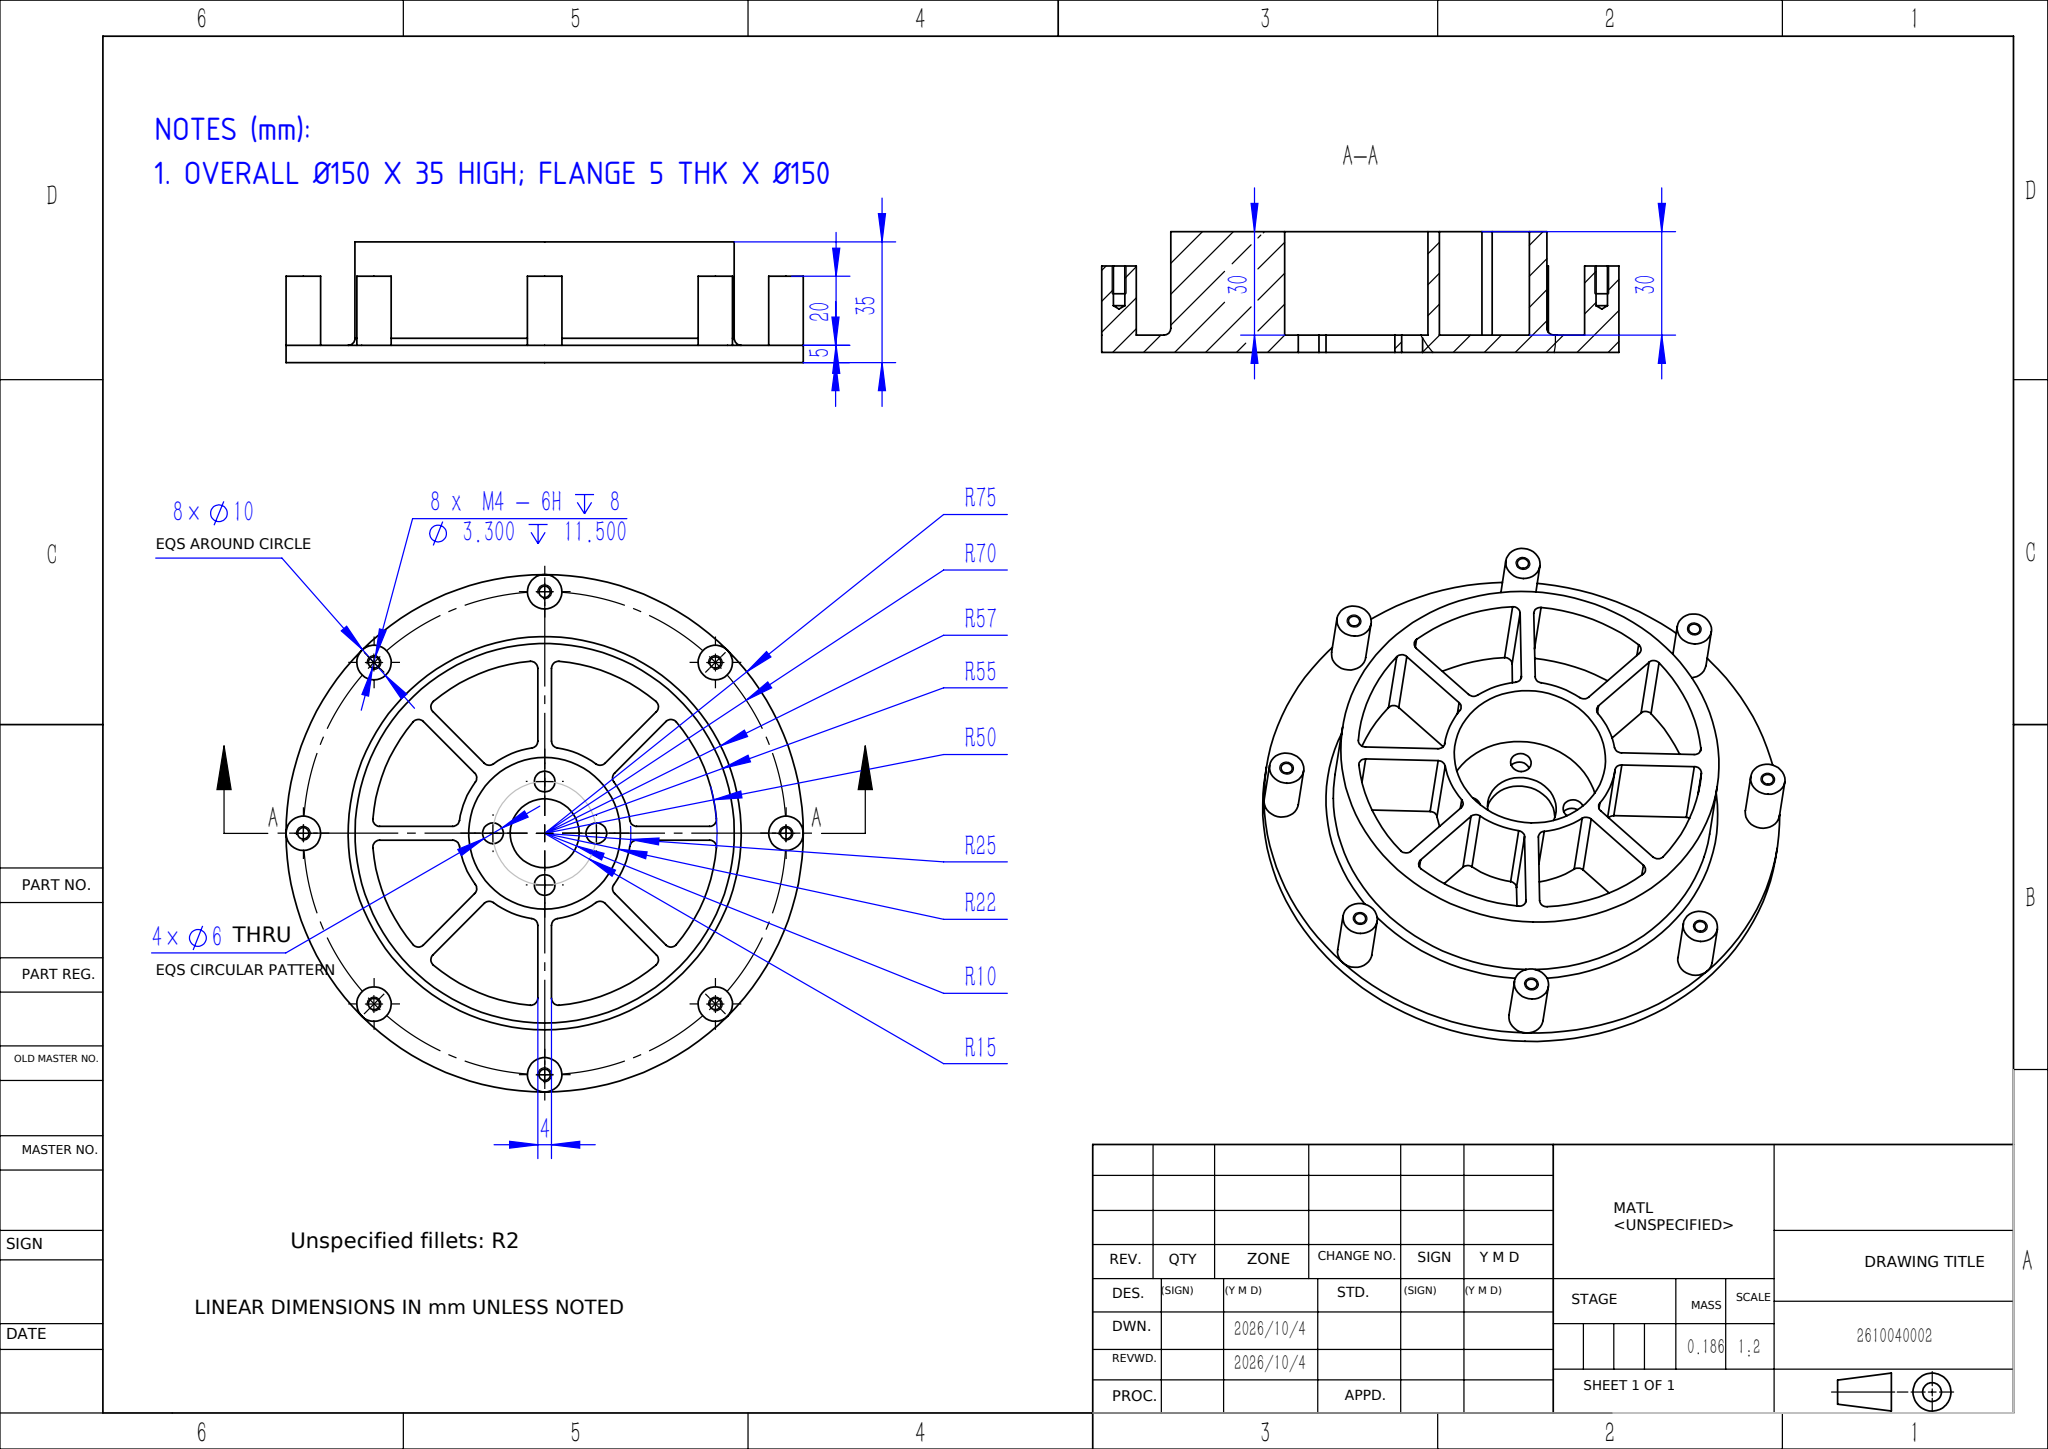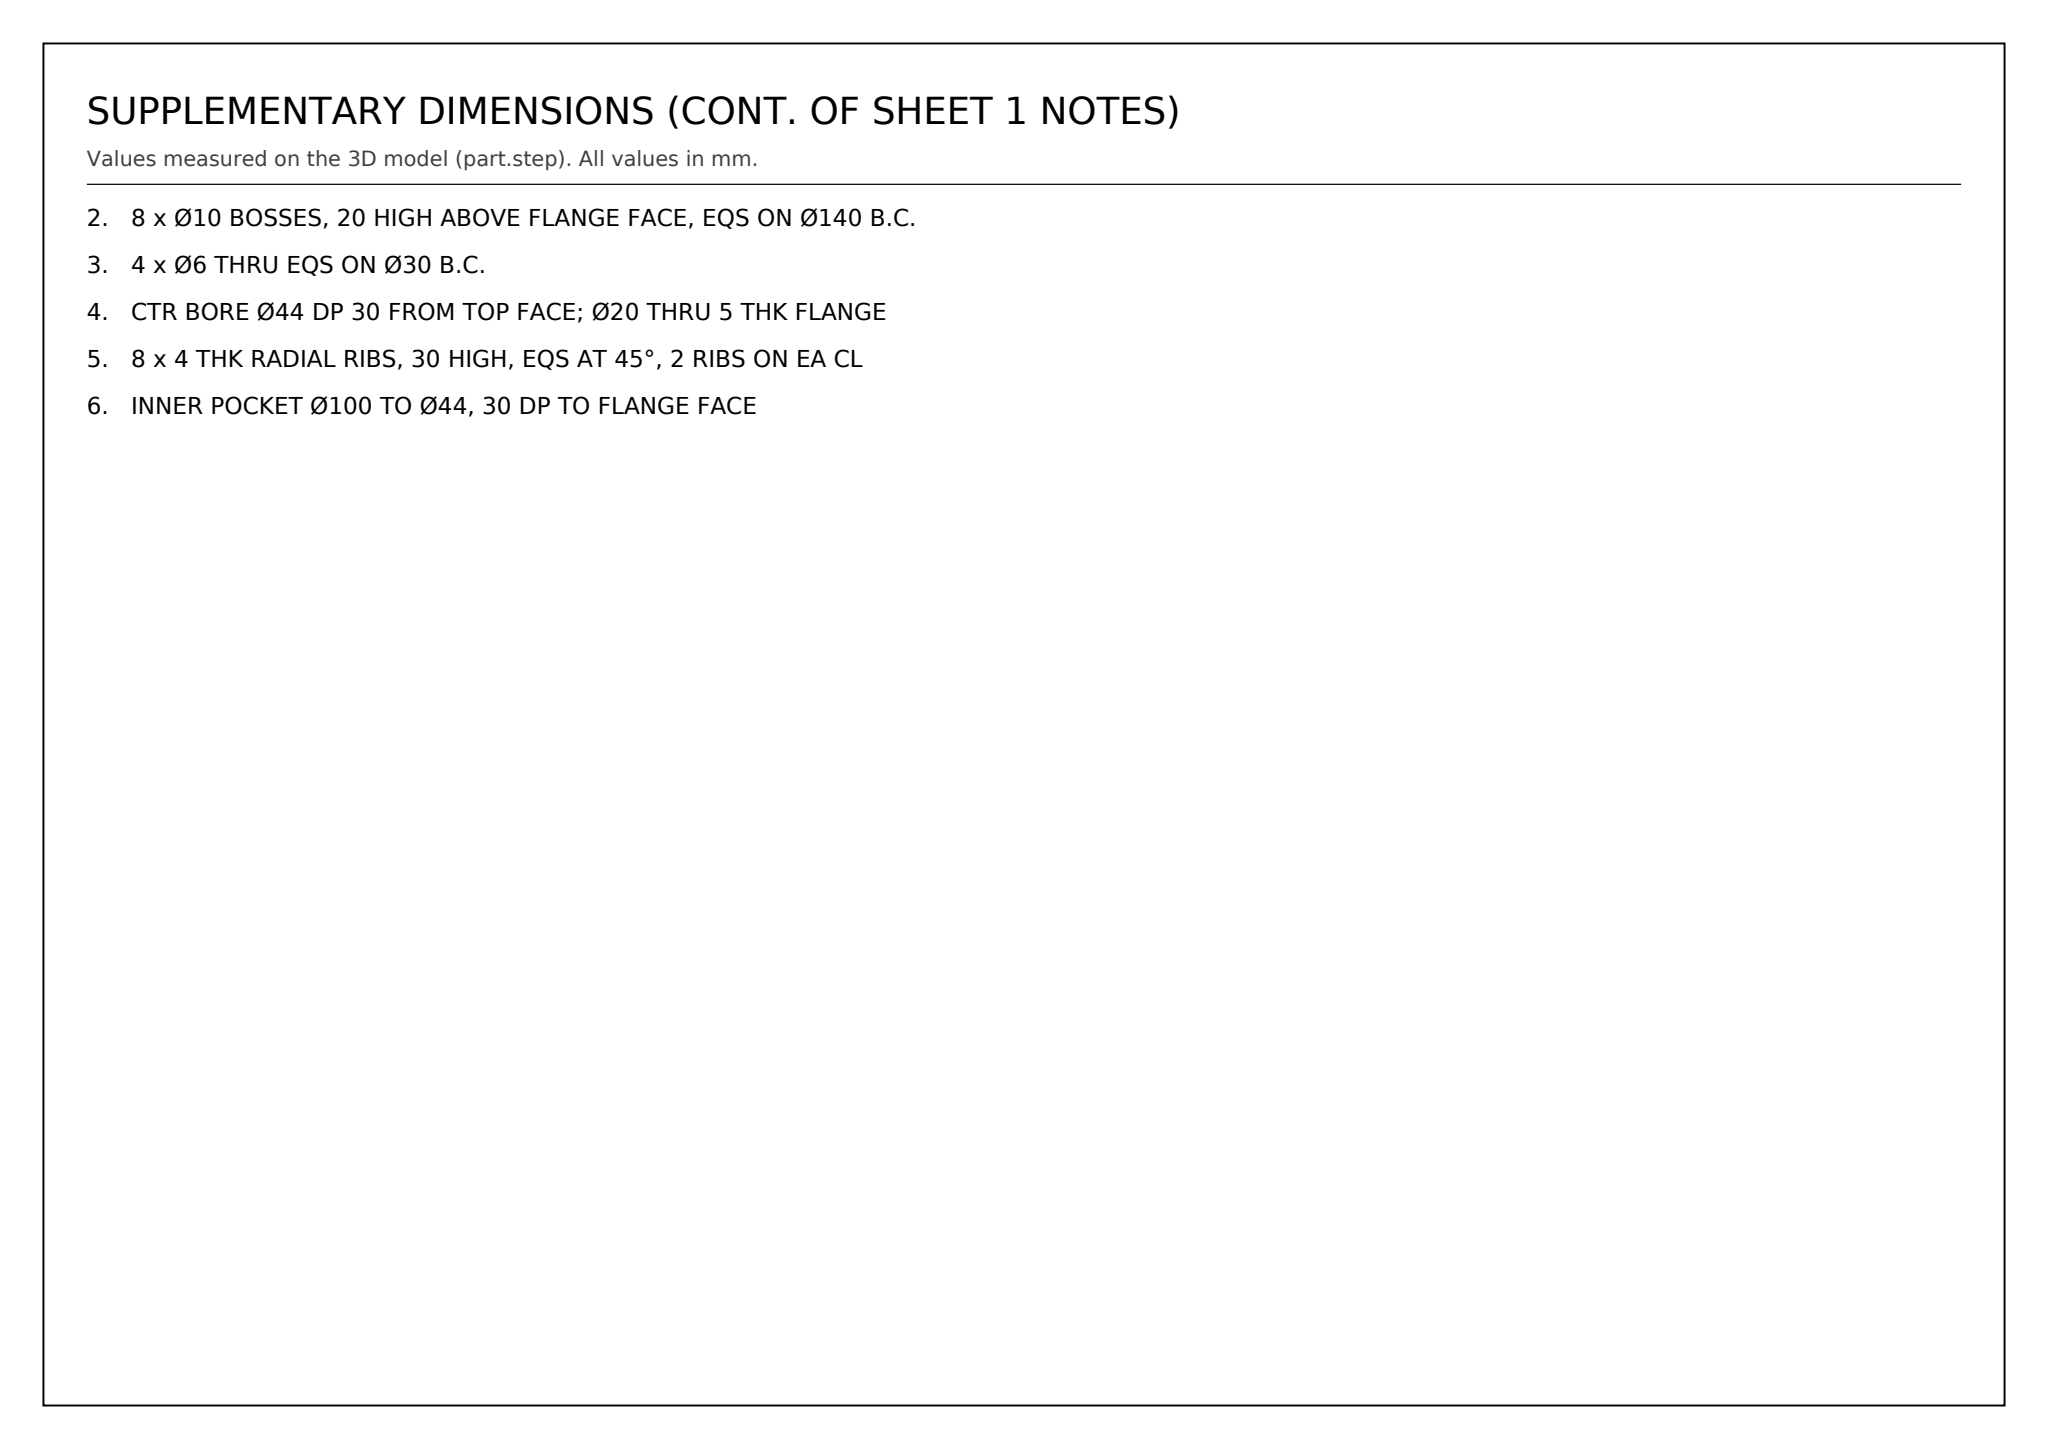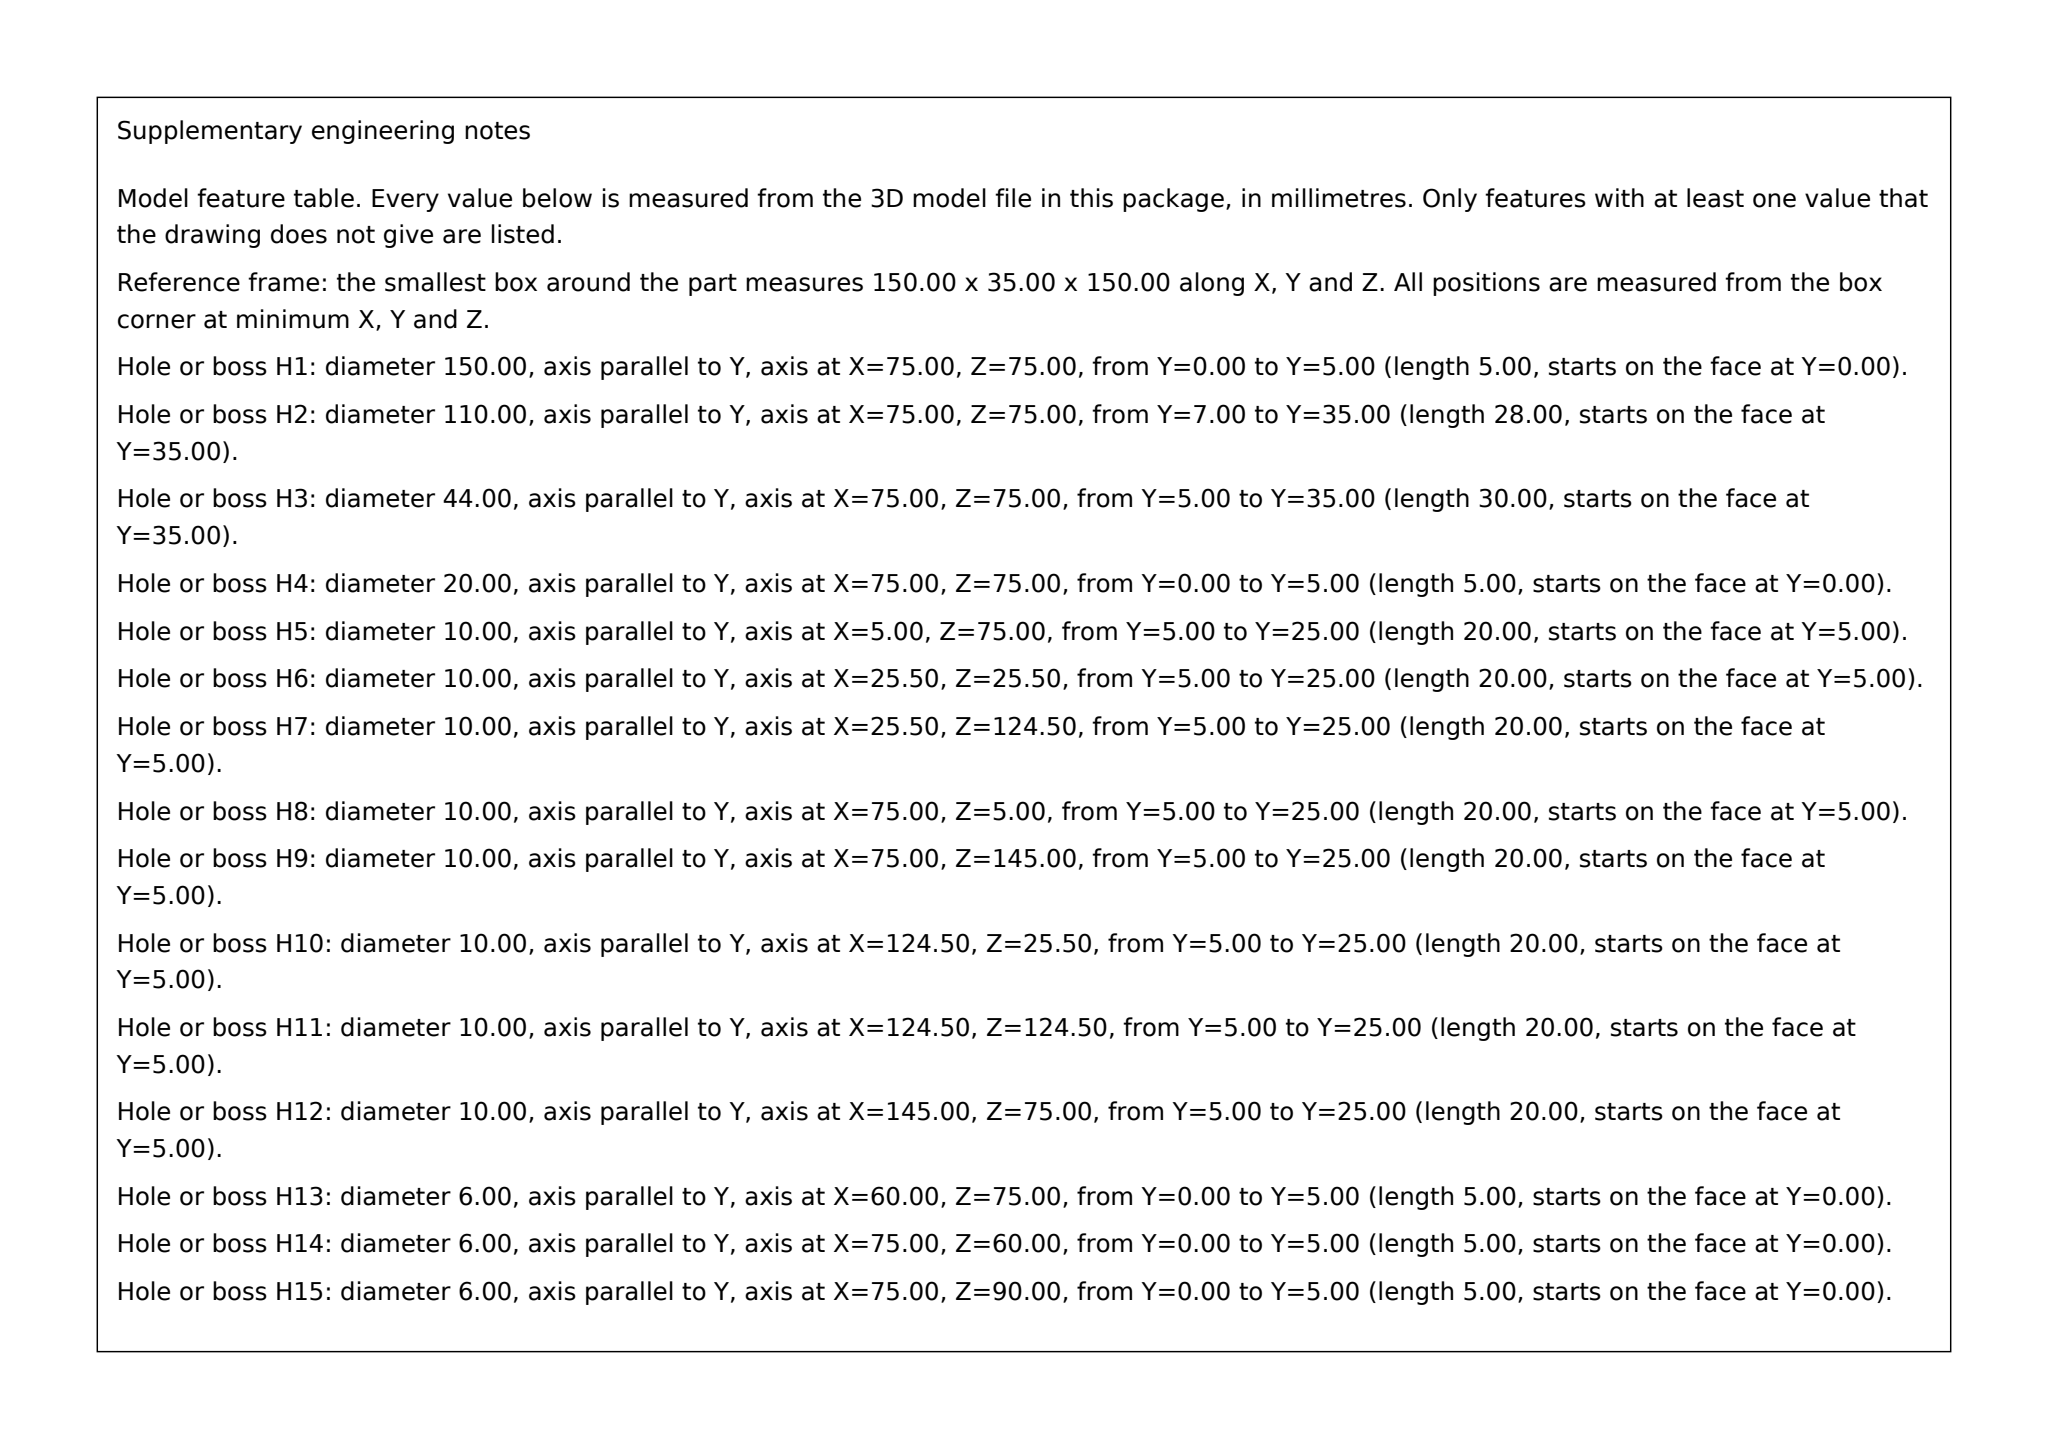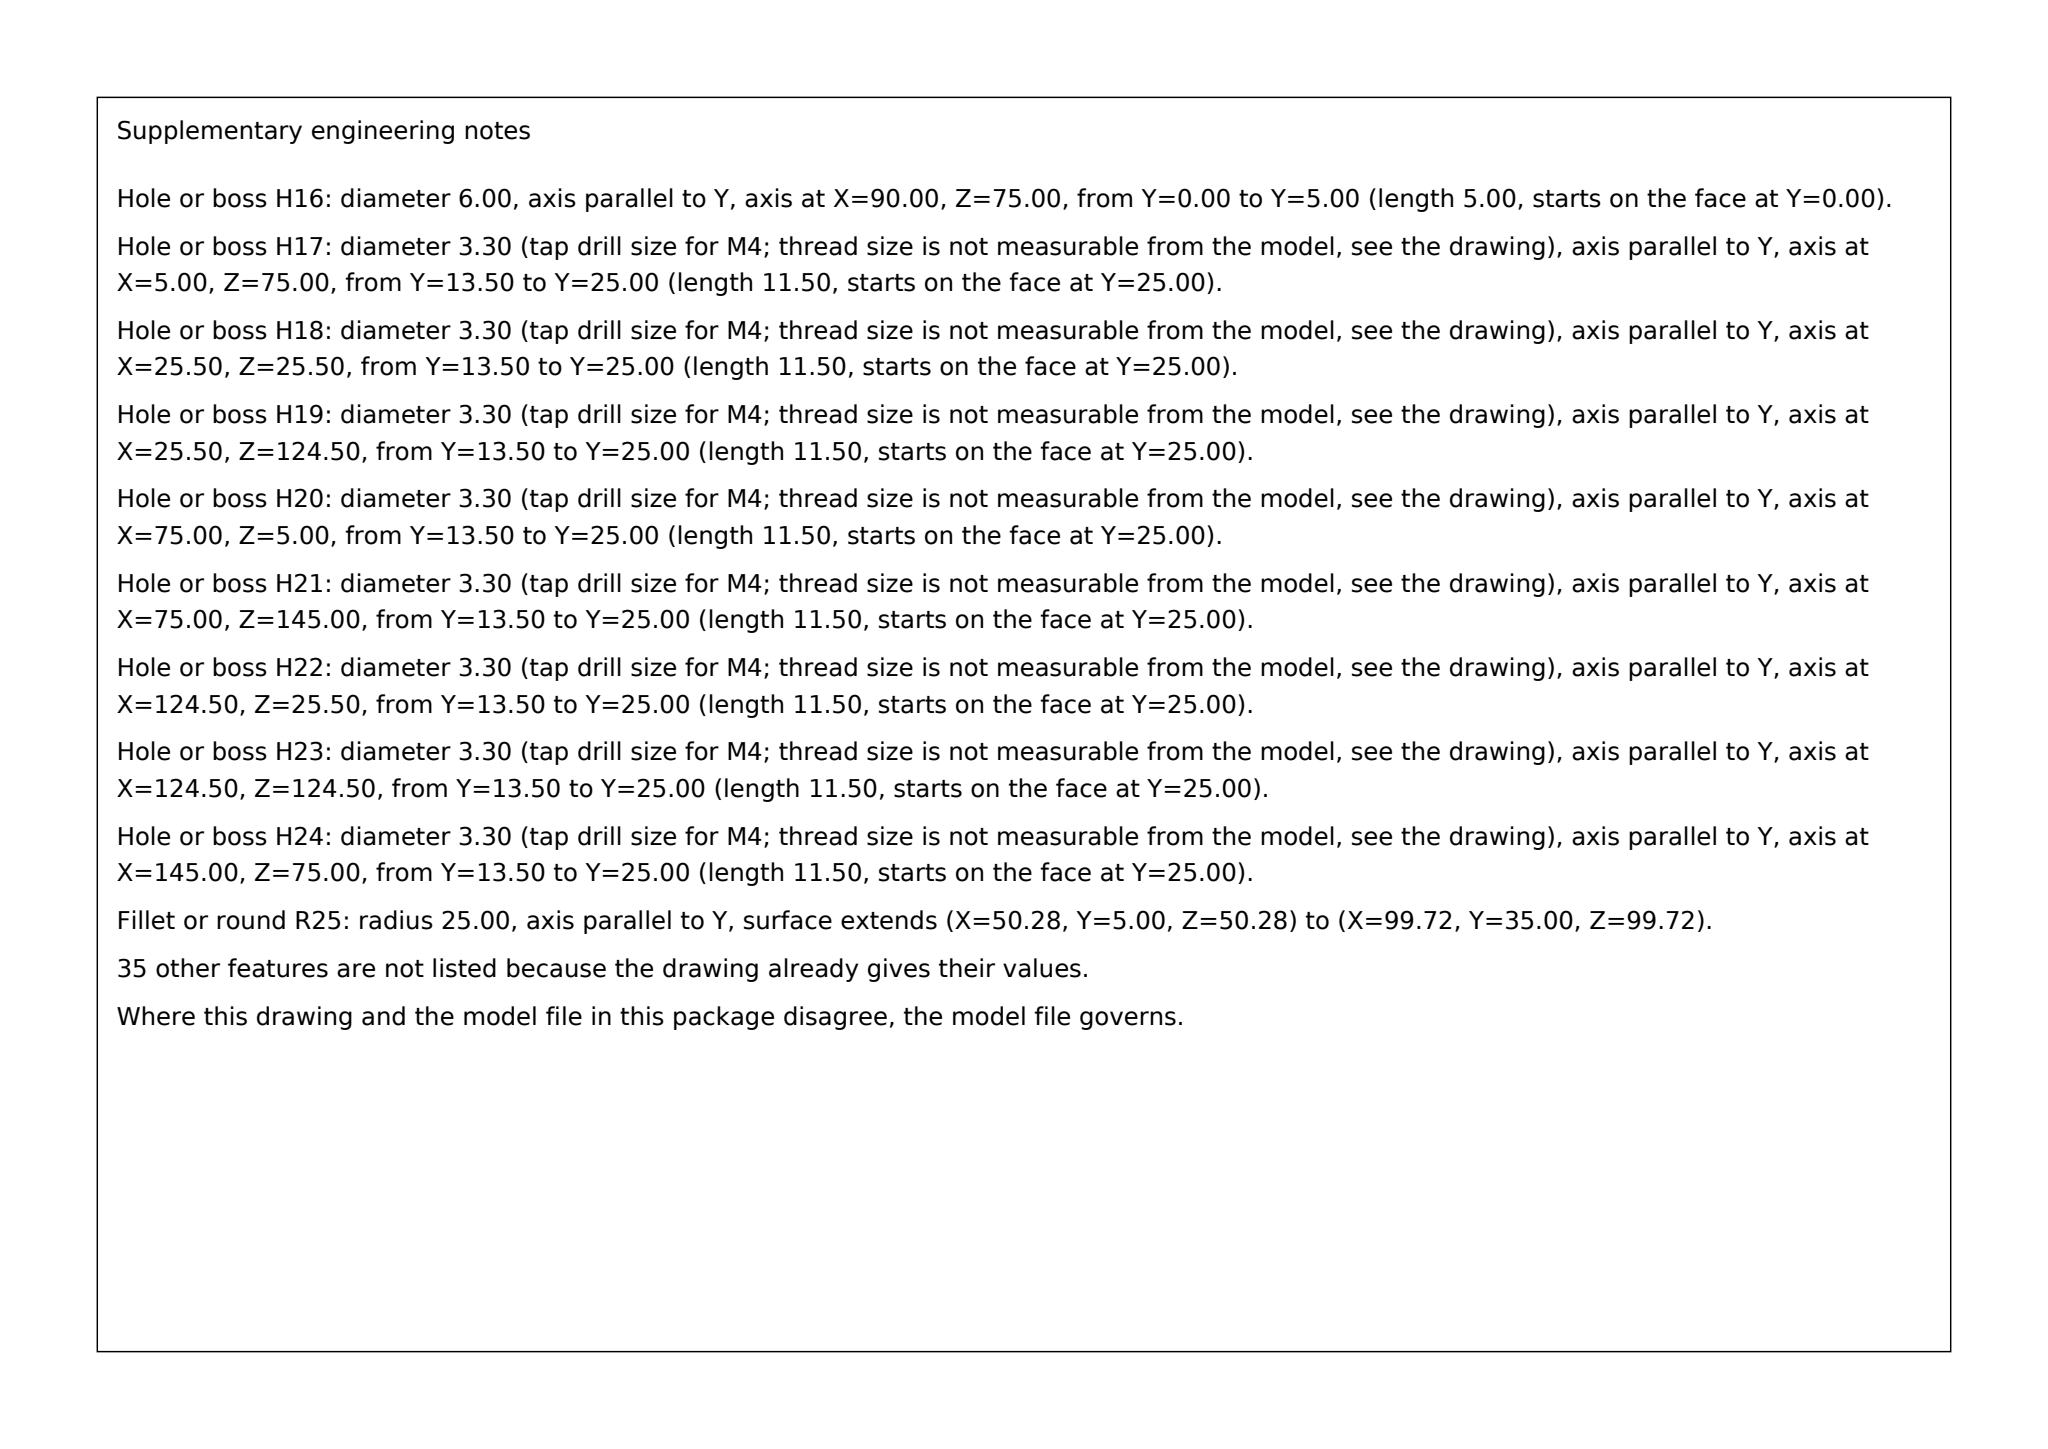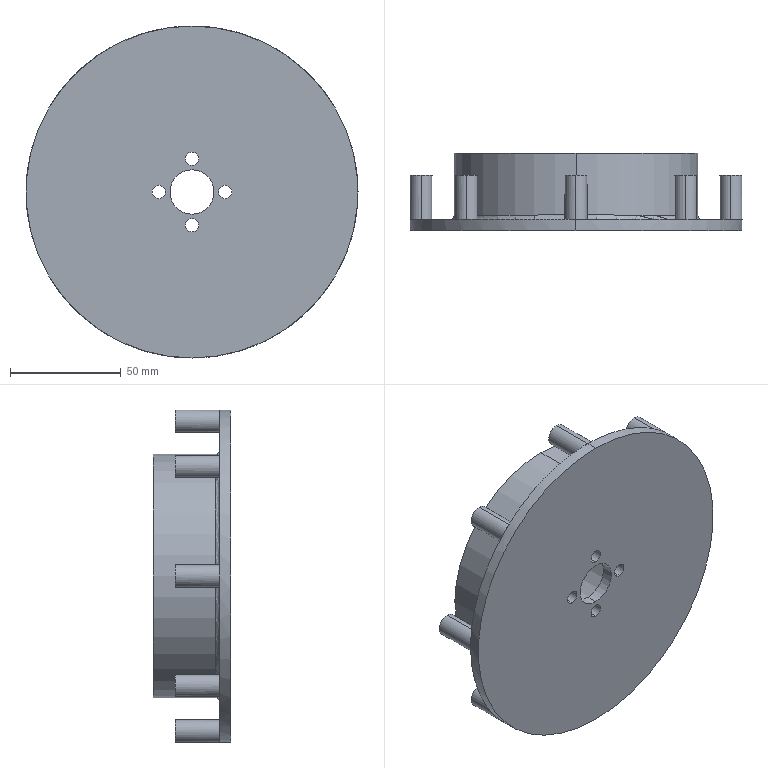Part | SolidWorks | mm | 1 solid | 156 faces | box 150 x 35 x 150 mm | volume 185846 mm3 | cylinder 102 | plane 36 | cone 16 | torus 2 | commonest cylinder face diameters 4 x38 3.3 x16 10 x16 6 x8 100 x8 50 x8 20 x2 44 x2
Drawing notes:
OVERALL Ø150 X 35 HIGH; FLANGE 5 THK X Ø150 | from the solid: Ø150 plate len 5 (y 0-5); overall planes y=0 to y=35
8 x Ø10 BOSSES, 20 HIGH ABOVE FLANGE FACE, EQS ON Ø140 B.C. | from the solid: Ø10 cyls len 20 between y=5 and y=25, r=70 from axis (75,75), 8 off at 45°
4 x Ø6 THRU EQS ON Ø30 B.C. | from the solid: Ø6 cyls at (60,75),(75,60),(75,90),(90,75), r=15 from (75,75)
CTR BORE Ø44 DP 30 FROM TOP FACE; Ø20 THRU 5 THK FLANGE | from the solid: Ø44 cyl len 30 (y=5-35) and Ø20 cyl len 5 (y=0-5), both on axis (75,75)
8 x 4 THK RADIAL RIBS, 30 HIGH, EQS AT 45°, 2 RIBS ON EA CL | from the solid: Rib faces x=73/77 & z=73/77 plus ribs at 45° increments, width 4, L=30
INNER POCKET Ø100 TO Ø44, 30 DP TO FLANGE FACE | from the solid: Pocket walls Ø100 & Ø44 len 30 from y=5 to y=35; plane y=5 = flange top face
build123d program:
from build123d import *

# Parameters (mm, degrees)
SKETCH1_R             = 75
BOSS_EXTRUDE1_DEPTH   = 5
SKETCH2_R             = 55
BOSS_EXTRUDE2_DEPTH   = 30
SHELL1_T              = -5
SKETCH3_R             = 25
SKETCH3_R_2           = 22
BOSS_EXTRUDE3_DEPTH   = 30
SKETCH4_W             = 4
SKETCH4_H             = 27.91
BOSS_EXTRUDE4_DEPTH   = 30
CIRPATTERN2_COUNT     = 8
SKETCH5_R             = 5
BOSS_EXTRUDE5_DEPTH   = 20
M4_TAPPED_HOLE1_D     = 3.3
M4_TAPPED_HOLE1_DEPTH = 11.5
M4_TAPPED_HOLE1_TIP   = 0.9914
SKETCH9_R             = 10
CUT_EXTRUDE1_DEPTH    = 111.227
FILLET1_R             = 2
SKETCH10_R            = 3
CUT_EXTRUDE2_DEPTH    = 111.227


with BuildPart() as part:
    # Sketch1 → Boss-Extrude1 (new body)
    with BuildSketch(Plane(origin=(0, 0, 0), x_dir=(1, 0, 0), z_dir=(0, 1, 0))):
        with Locations(Location((0, 0, 0), (0, 0, 270))):
            Circle(SKETCH1_R)
    extrude(amount=BOSS_EXTRUDE1_DEPTH)

    # Sketch2 → Boss-Extrude2 (add)
    with BuildSketch(Plane(origin=(0, 5, 0), x_dir=(1, 0, 0), z_dir=(0, 1, 0))):
        with Locations(Location((0, 0, 0), (0, 0, 270))):
            Circle(SKETCH2_R)
    extrude(amount=BOSS_EXTRUDE2_DEPTH)

    # Shell1
    shell1_openings = [part.faces().sort_by_distance(p)[0] for p in [
        (0, 35, 0),
    ]]
    offset(amount=SHELL1_T, openings=shell1_openings, kind=Kind.INTERSECTION)

    # Sketch3 → Boss-Extrude3 (add)
    with BuildSketch(Plane(origin=(0, 5, 0), x_dir=(1, 0, 0), z_dir=(0, 1, 0))):
        with Locations(Location((0, 0, 0), (0, 0, 270))):
            Circle(SKETCH3_R)
        with Locations(Location((0, 0, 0), (0, 0, 270))):
            Circle(SKETCH3_R_2, mode=Mode.SUBTRACT)
    extrude(amount=BOSS_EXTRUDE3_DEPTH)

    # Sketch4 → Boss-Extrude4 (add)
    with BuildSketch(Plane(origin=(0, 5, 0), x_dir=(1, 0, 0), z_dir=(0, 1, 0))):
        with Locations((0, 37.312)):
            Rectangle(SKETCH4_W, SKETCH4_H)
    boss_extrude4 = extrude(amount=BOSS_EXTRUDE4_DEPTH)

    # CirPattern2: Boss-Extrude4 ×8 about axis
    cirpattern2_axis = Axis((0, 0, 0), (0, 1, 0))
    for i in range(1, CIRPATTERN2_COUNT):
        add(boss_extrude4.rotate(cirpattern2_axis, i * 360 / CIRPATTERN2_COUNT))

    # Sketch5 → Boss-Extrude5 (add)
    with BuildSketch(Plane(origin=(0, 5, 0), x_dir=(1, 0, 0), z_dir=(0, 1, 0))):
        with Locations(Location((0, 70, 0), (0, 0, 90))):
            Circle(SKETCH5_R)
        with Locations(Location((49.497, 49.497, 0), (0, 0, 45))):
            Circle(SKETCH5_R)
        with Locations(Location((70, 0, 0), (0, 0, 360))):
            Circle(SKETCH5_R)
        with Locations(Location((49.497, -49.497, 0), (0, 0, 315))):
            Circle(SKETCH5_R)
        with Locations(Location((0, -70, 0), (0, 0, 270))):
            Circle(SKETCH5_R)
        with Locations(Location((-49.497, -49.497, 0), (0, 0, 225))):
            Circle(SKETCH5_R)
        with Locations(Location((-70, 0, 0), (0, 0, 180))):
            Circle(SKETCH5_R)
        with Locations(Location((-49.497, 49.497, 0), (0, 0, 135))):
            Circle(SKETCH5_R)
    extrude(amount=BOSS_EXTRUDE5_DEPTH)

    # M4 Tapped Hole1
    with Locations(Plane(origin=(0, 25, 0), x_dir=(1, 0, 0), z_dir=(0, 1, 0))):
        with Locations((0, 70), (49.497, 49.497), (70, 0), (49.497, -49.497), (0, -70), (-49.497, -49.497), (-70, 0), (-49.497, 49.497)):
            Hole(M4_TAPPED_HOLE1_D / 2, depth=M4_TAPPED_HOLE1_DEPTH)
            with Locations((0, 0, -(M4_TAPPED_HOLE1_DEPTH + M4_TAPPED_HOLE1_TIP / 2))):  # 118° drill point
                Cone(0, M4_TAPPED_HOLE1_D / 2, M4_TAPPED_HOLE1_TIP, mode=Mode.SUBTRACT)

    # Sketch9 → Cut-Extrude1 (cut, through all)
    with BuildSketch(Plane(origin=(0, 5, 0), x_dir=(1, 0, 0), z_dir=(0, 1, 0))):
        with Locations(Location((0, 0, 0), (0, 0, 270))):
            Circle(SKETCH9_R)
    extrude(amount=-CUT_EXTRUDE1_DEPTH, mode=Mode.SUBTRACT)

    # Fillet1
    fillet1_edges = [part.edges().sort_by_distance(p)[0] for p in [
        (-49.96, 20, 2),
        (-24.92, 20, 2),
        (-49.96, 20, -2),
        (-24.92, 20, -2),
        (-33.913, 20, 36.741),
        (-16.207, 20, 19.035),
        (-36.741, 20, 33.913),
        (-19.035, 20, 16.207),
        (2, 20, 49.96),
        (2, 20, 24.92),
        (-2, 20, 49.96),
        (-2, 20, 24.92),
        (36.741, 20, 33.913),
        (19.035, 20, 16.207),
        (33.913, 20, 36.741),
        (16.207, 20, 19.035),
        (49.96, 20, -2),
        (24.92, 20, -2),
        (49.96, 20, 2),
        (24.92, 20, 2),
        (33.913, 20, -36.741),
        (16.207, 20, -19.035),
        (36.741, 20, -33.913),
        (19.035, 20, -16.207),
        (-36.741, 20, -33.913),
        (-19.035, 20, -16.207),
        (-33.913, 20, -36.741),
        (-16.207, 20, -19.035),
        (2, 20, -24.92),
        (-2, 20, -24.92),
        (-2, 20, -49.96),
        (2, 20, -49.96),
        (0, 5, -55),
    ]]
    fillet(fillet1_edges, radius=FILLET1_R)

    # Sketch10 → Cut-Extrude2 (cut, through all)
    with BuildSketch(Plane(origin=(0, 5, 0), x_dir=(1, 0, 0), z_dir=(0, 1, 0))):
        with Locations(Location((0, 15, 0), (0, 0, 270))):
            Circle(SKETCH10_R)
        with Locations(Location((15, 0, 0), (0, 0, 270))):
            Circle(SKETCH10_R)
        with Locations(Location((0, -15, 0), (0, 0, 270))):
            Circle(SKETCH10_R)
        with Locations(Location((-15, 0, 0), (0, 0, 270))):
            Circle(SKETCH10_R)
    extrude(amount=-CUT_EXTRUDE2_DEPTH, mode=Mode.SUBTRACT)


solid = part.part